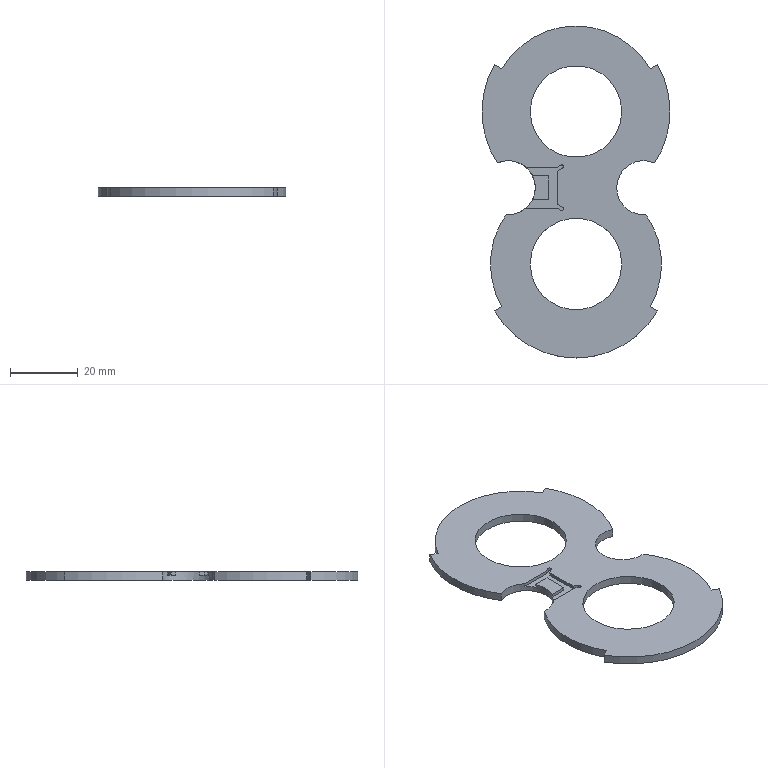Component | NX | CLYB_03_WEARPLATE_2 | 1 solid | 30 faces | volume 7345 mm3 | plane 18 | cylinder 12 | commonest cylinder face diameters 55.5 x3 50.5 x3 16 x2 27 x2 1 x2